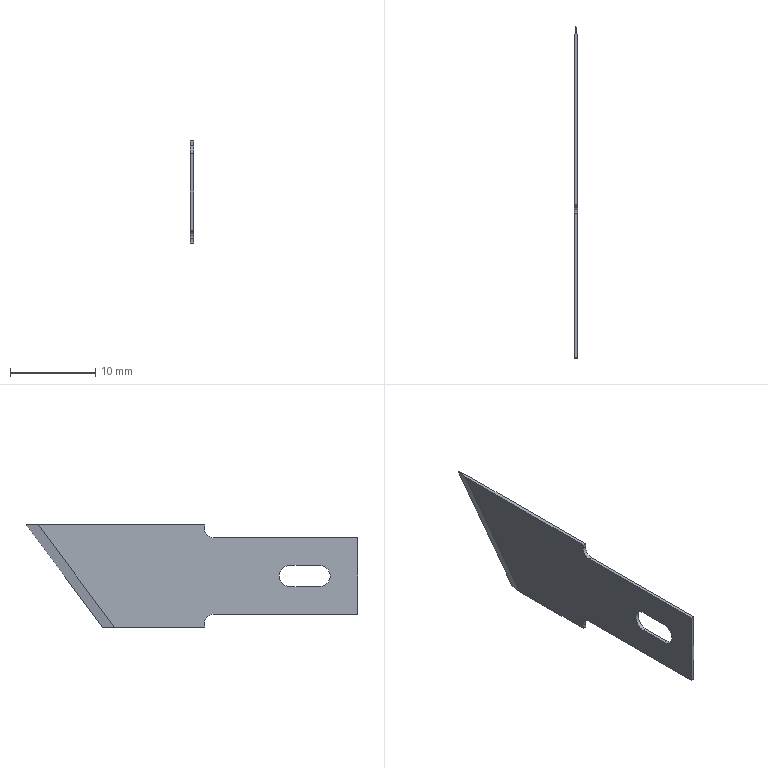Component | SolidWorks | 20#EngravingKnifeBlade-2 | 1 solid | 17 faces | volume 135 mm3 | plane 13 | cylinder 4 | commonest cylinder face diameters 2.5 x2 2 x2